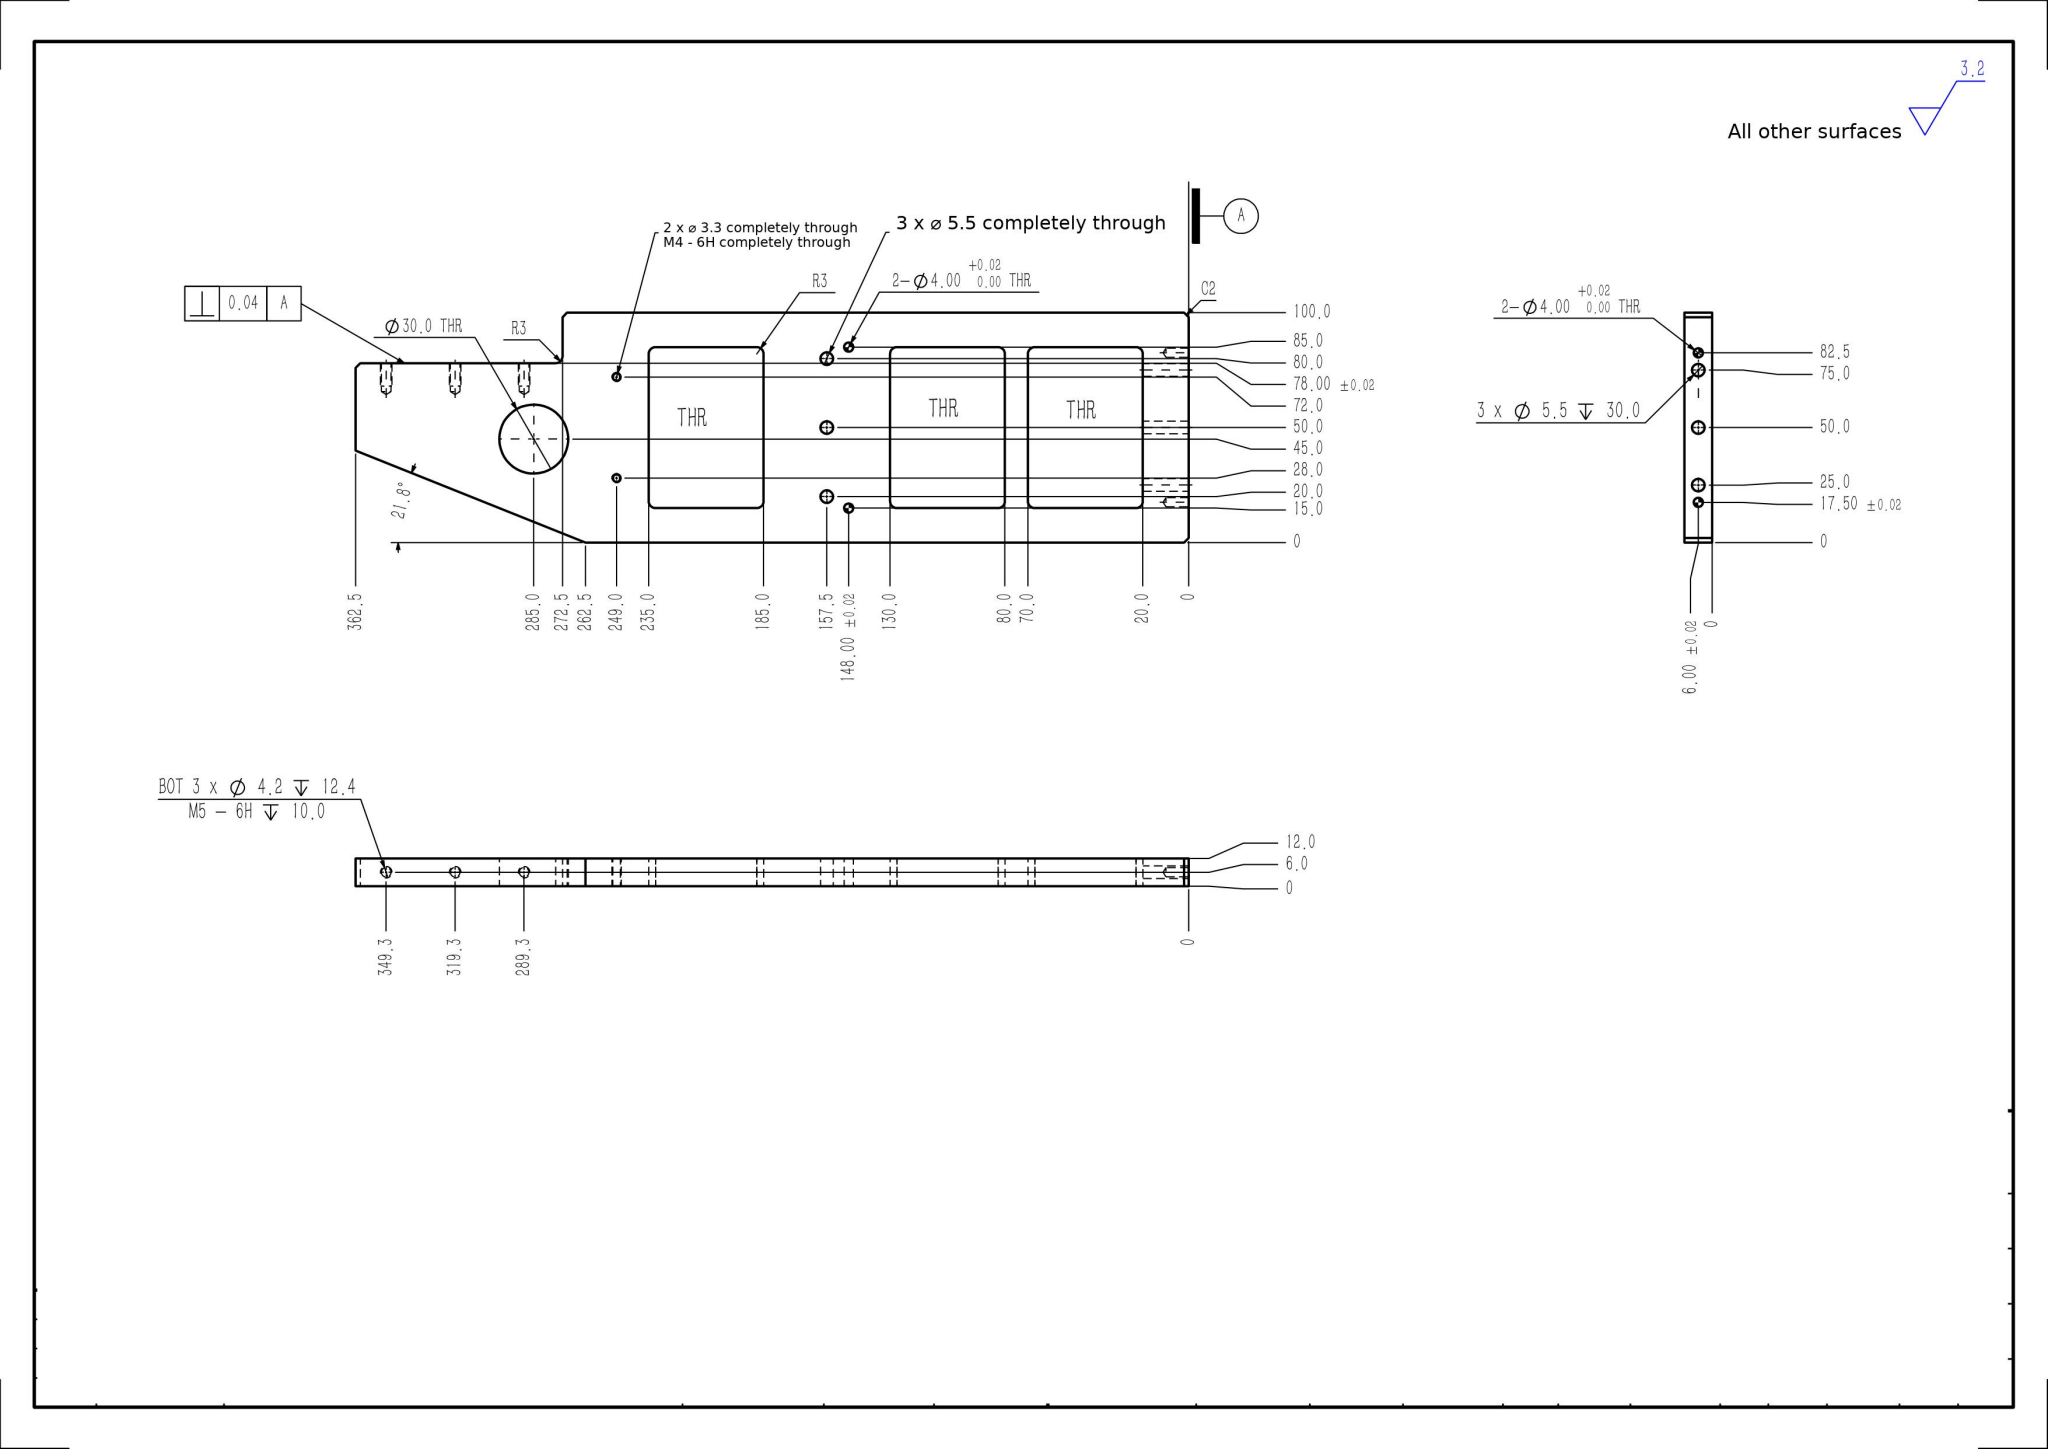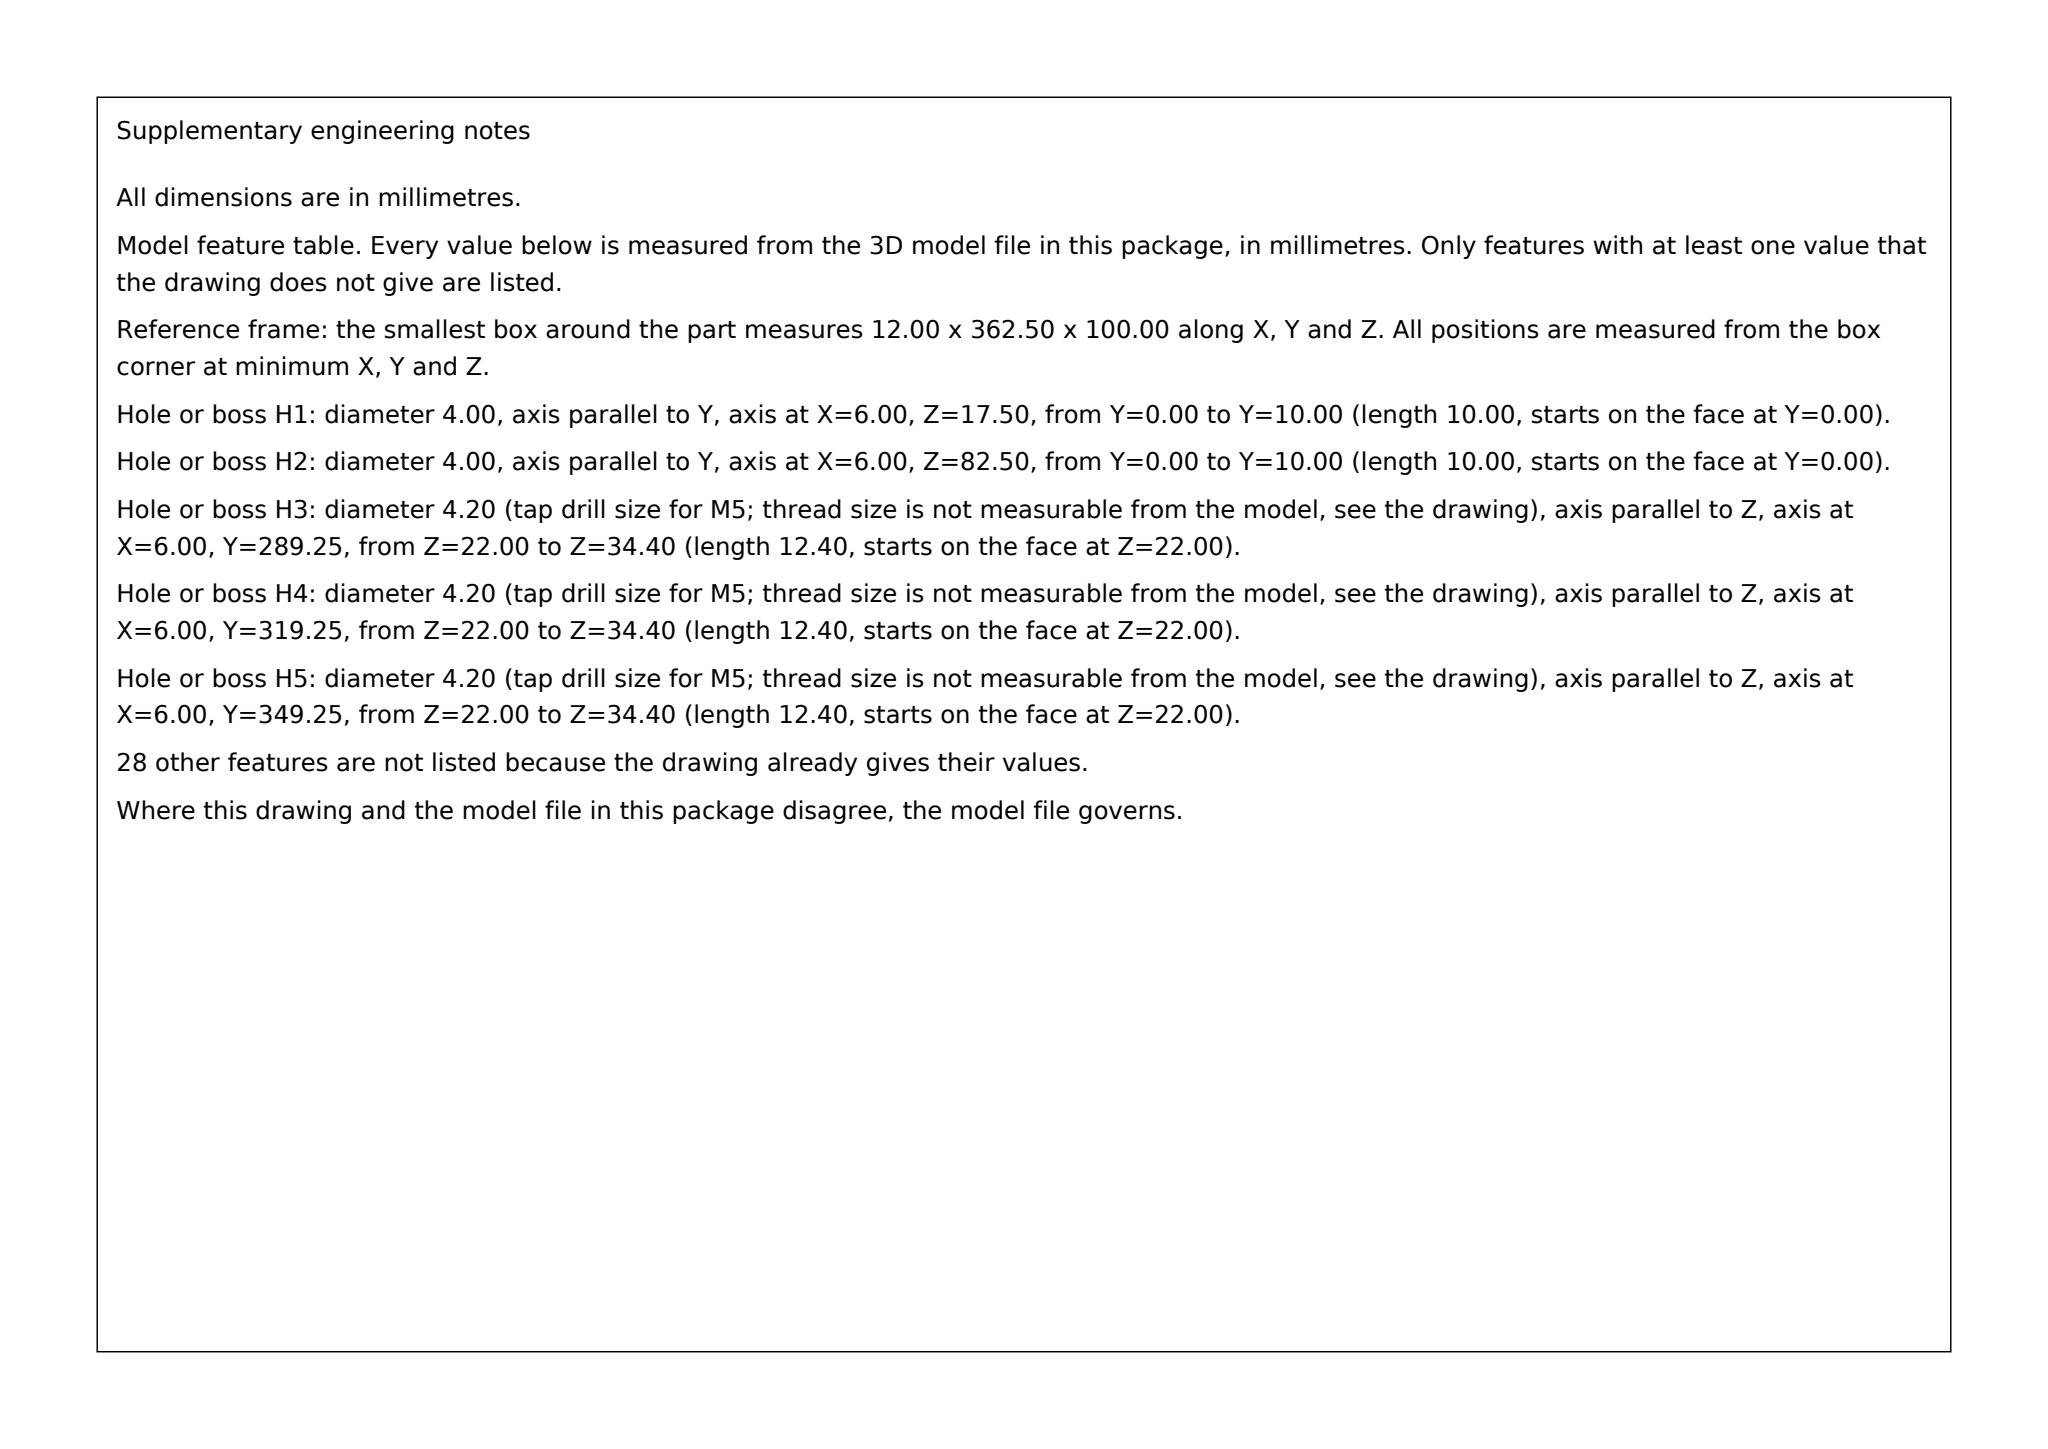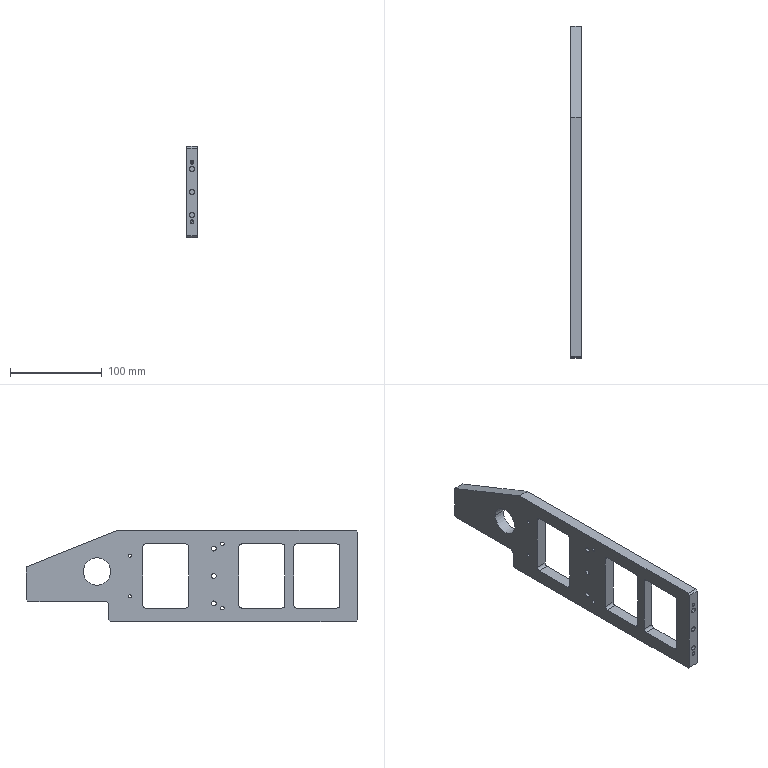Part | SolidWorks | mm | 1 solid | 80 faces | box 12 x 362.5 x 100 mm | volume 249381 mm3 | cylinder 45 | plane 25 | cone 10 | commonest cylinder face diameters 6 x13 5.5 x12 4 x8 4.2 x6 3.3 x4 30 x2
build123d program:
from build123d import *

# Parameters (mm, degrees)
BOSS_EXTRUDE1_DEPTH            = 6
SKETCH15_W                     = 55.085
SKETCH15_H                     = 186.51
CUT_EXTRUDE2_DEPTH             = 367.129
SKETCH2_R                      = 15
SKETCH2_W                      = 50
SKETCH2_H                      = 70
CUT_EXTRUDE1_DEPTH             = 367.129
FILLET1_R                      = 3
F_5_5_5_5_DIAMETER_HOLE2_D     = 5.5
F_5_5_5_5_DIAMETER_HOLE2_DEPTH = 30
F_5_5_5_5_DIAMETER_HOLE2_TIP   = 1.652
SIZE_MM_DOWEL_PIN_HOLE_1_D     = 4
SIZE_MM_DOWEL_PIN_HOLE_1_DEPTH = 10
SIZE_MM_DOWEL_PIN_HOLE_1_TIP   = 1.202
M5_TAPPED_HOLE1_D              = 4.2
M5_TAPPED_HOLE1_DEPTH          = 12.4
M5_TAPPED_HOLE1_TIP            = 1.262
F_5_5_5_5_DIAMETER_HOLE1_D     = 5.5
SIZE_MM_DOWEL_PIN_HOLE_2_D     = 4
CHAMFER1_SIZE                  = 2
M4_TAPPED_HOLE1_D              = 3.3


with BuildPart() as part:
    # Sketch1 → Boss-Extrude1 (new, symmetric)
    with BuildSketch(Plane(origin=(0, 0, 0), x_dir=(0, -1, 0), z_dir=(1, 0, 0))):
        Polygon((0, 50), (-362.5, 50), (-362.5, -10), (-262.5, -50), (0, -50), align=None)
    extrude(amount=BOSS_EXTRUDE1_DEPTH, both=True)

    # Sketch15 → Cut-Extrude2 (cut, through all)
    with BuildSketch(Plane(origin=(6, 0, 0), x_dir=(0, 0, -1), z_dir=(1, 0, 0))):
        with Locations((55.542, 365.755)):
            Rectangle(SKETCH15_W, SKETCH15_H)
    extrude(amount=-CUT_EXTRUDE2_DEPTH, mode=Mode.SUBTRACT)

    # Sketch2 → Cut-Extrude1 (cut, through all)
    with BuildSketch(Plane(origin=(6, 0, 0), x_dir=(0, -1, 0), z_dir=(1, 0, 0))):
        with Locations(Location((-285, -5, 0), (0, 0, 180))):
            Circle(SKETCH2_R)
        with Locations((-45, 0)):
            Rectangle(SKETCH2_W, SKETCH2_H)
        with Locations((-105, 0)):
            Rectangle(SKETCH2_W, SKETCH2_H)
        with Locations((-210, 0)):
            Rectangle(SKETCH2_W, SKETCH2_H)
    extrude(amount=-CUT_EXTRUDE1_DEPTH, mode=Mode.SUBTRACT)

    # Fillet1
    fillet1_edges = [part.edges().sort_by_distance(p)[0] for p in [
        (0, 272.5, -28),
        (0, 70, 35),
        (0, 70, -35),
        (0, 20, -35),
        (0, 20, 35),
        (0, 130, 35),
        (0, 130, -35),
        (0, 80, -35),
        (0, 80, 35),
        (0, 235, 35),
        (0, 235, -35),
        (0, 185, -35),
        (0, 185, 35),
    ]]
    fillet(fillet1_edges, radius=FILLET1_R)

    # 5.5 _5.5_ Diameter Hole2
    with Locations(Plane(origin=(0, 0, 0), x_dir=(0, 0, -1), z_dir=(0, -1, 0))):
        with Locations((-25, 0), (25, 0), (0, 0)):
            Hole(F_5_5_5_5_DIAMETER_HOLE2_D / 2, depth=F_5_5_5_5_DIAMETER_HOLE2_DEPTH)
            with Locations((0, 0, -(F_5_5_5_5_DIAMETER_HOLE2_DEPTH + F_5_5_5_5_DIAMETER_HOLE2_TIP / 2))):  # 118° drill point
                Cone(0, F_5_5_5_5_DIAMETER_HOLE2_D / 2, F_5_5_5_5_DIAMETER_HOLE2_TIP, mode=Mode.SUBTRACT)

    # Size mm Dowel Pin Hole 1
    with Locations(Plane(origin=(0, 0, 0), x_dir=(0, 0, -1), z_dir=(0, -1, 0))):
        with Locations((-32.5, 0), (32.5, 0)):
            Hole(SIZE_MM_DOWEL_PIN_HOLE_1_D / 2, depth=SIZE_MM_DOWEL_PIN_HOLE_1_DEPTH)
            with Locations((0, 0, -(SIZE_MM_DOWEL_PIN_HOLE_1_DEPTH + SIZE_MM_DOWEL_PIN_HOLE_1_TIP / 2))):  # 118° drill point
                Cone(0, SIZE_MM_DOWEL_PIN_HOLE_1_D / 2, SIZE_MM_DOWEL_PIN_HOLE_1_TIP, mode=Mode.SUBTRACT)

    # M5 Tapped Hole1
    with Locations(Plane(origin=(0, 0, -28), x_dir=(-1, 0, 0), z_dir=(0, 0, -1))):
        with Locations((0, 349.25), (0, 319.25), (0, 289.25)):
            Hole(M5_TAPPED_HOLE1_D / 2, depth=M5_TAPPED_HOLE1_DEPTH)
            with Locations((0, 0, -(M5_TAPPED_HOLE1_DEPTH + M5_TAPPED_HOLE1_TIP / 2))):  # 118° drill point
                Cone(0, M5_TAPPED_HOLE1_D / 2, M5_TAPPED_HOLE1_TIP, mode=Mode.SUBTRACT)

    # 5.5 _5.5_ Diameter Hole1 (through all)
    with Locations(Plane.ZY.offset(6)):
        with Locations((30, 157.5), (0, 157.5), (-30, 157.5)):
            Hole(F_5_5_5_5_DIAMETER_HOLE1_D / 2)

    # Size mm Dowel Pin Hole 2 (through all)
    with Locations(Plane(origin=(6, 0, 0), x_dir=(0, 0, -1), z_dir=(1, 0, 0))):
        with Locations((-35, 148), (35, 148)):
            Hole(SIZE_MM_DOWEL_PIN_HOLE_2_D / 2)

    # Chamfer1
    chamfer1_edges = [part.edges().sort_by_distance(p)[0] for p in [
        (0, 362.5, -28),
        (0, 272.5, -50),
        (0, 0, 50),
        (0, 0, -50),
    ]]
    chamfer(chamfer1_edges, length=CHAMFER1_SIZE)

    # M4 Tapped Hole1 (through all)
    with Locations(Plane(origin=(6, 0, 0), x_dir=(0, 0, -1), z_dir=(1, 0, 0))):
        with Locations((-22, 249), (22, 249)):
            Hole(M4_TAPPED_HOLE1_D / 2)


solid = part.part